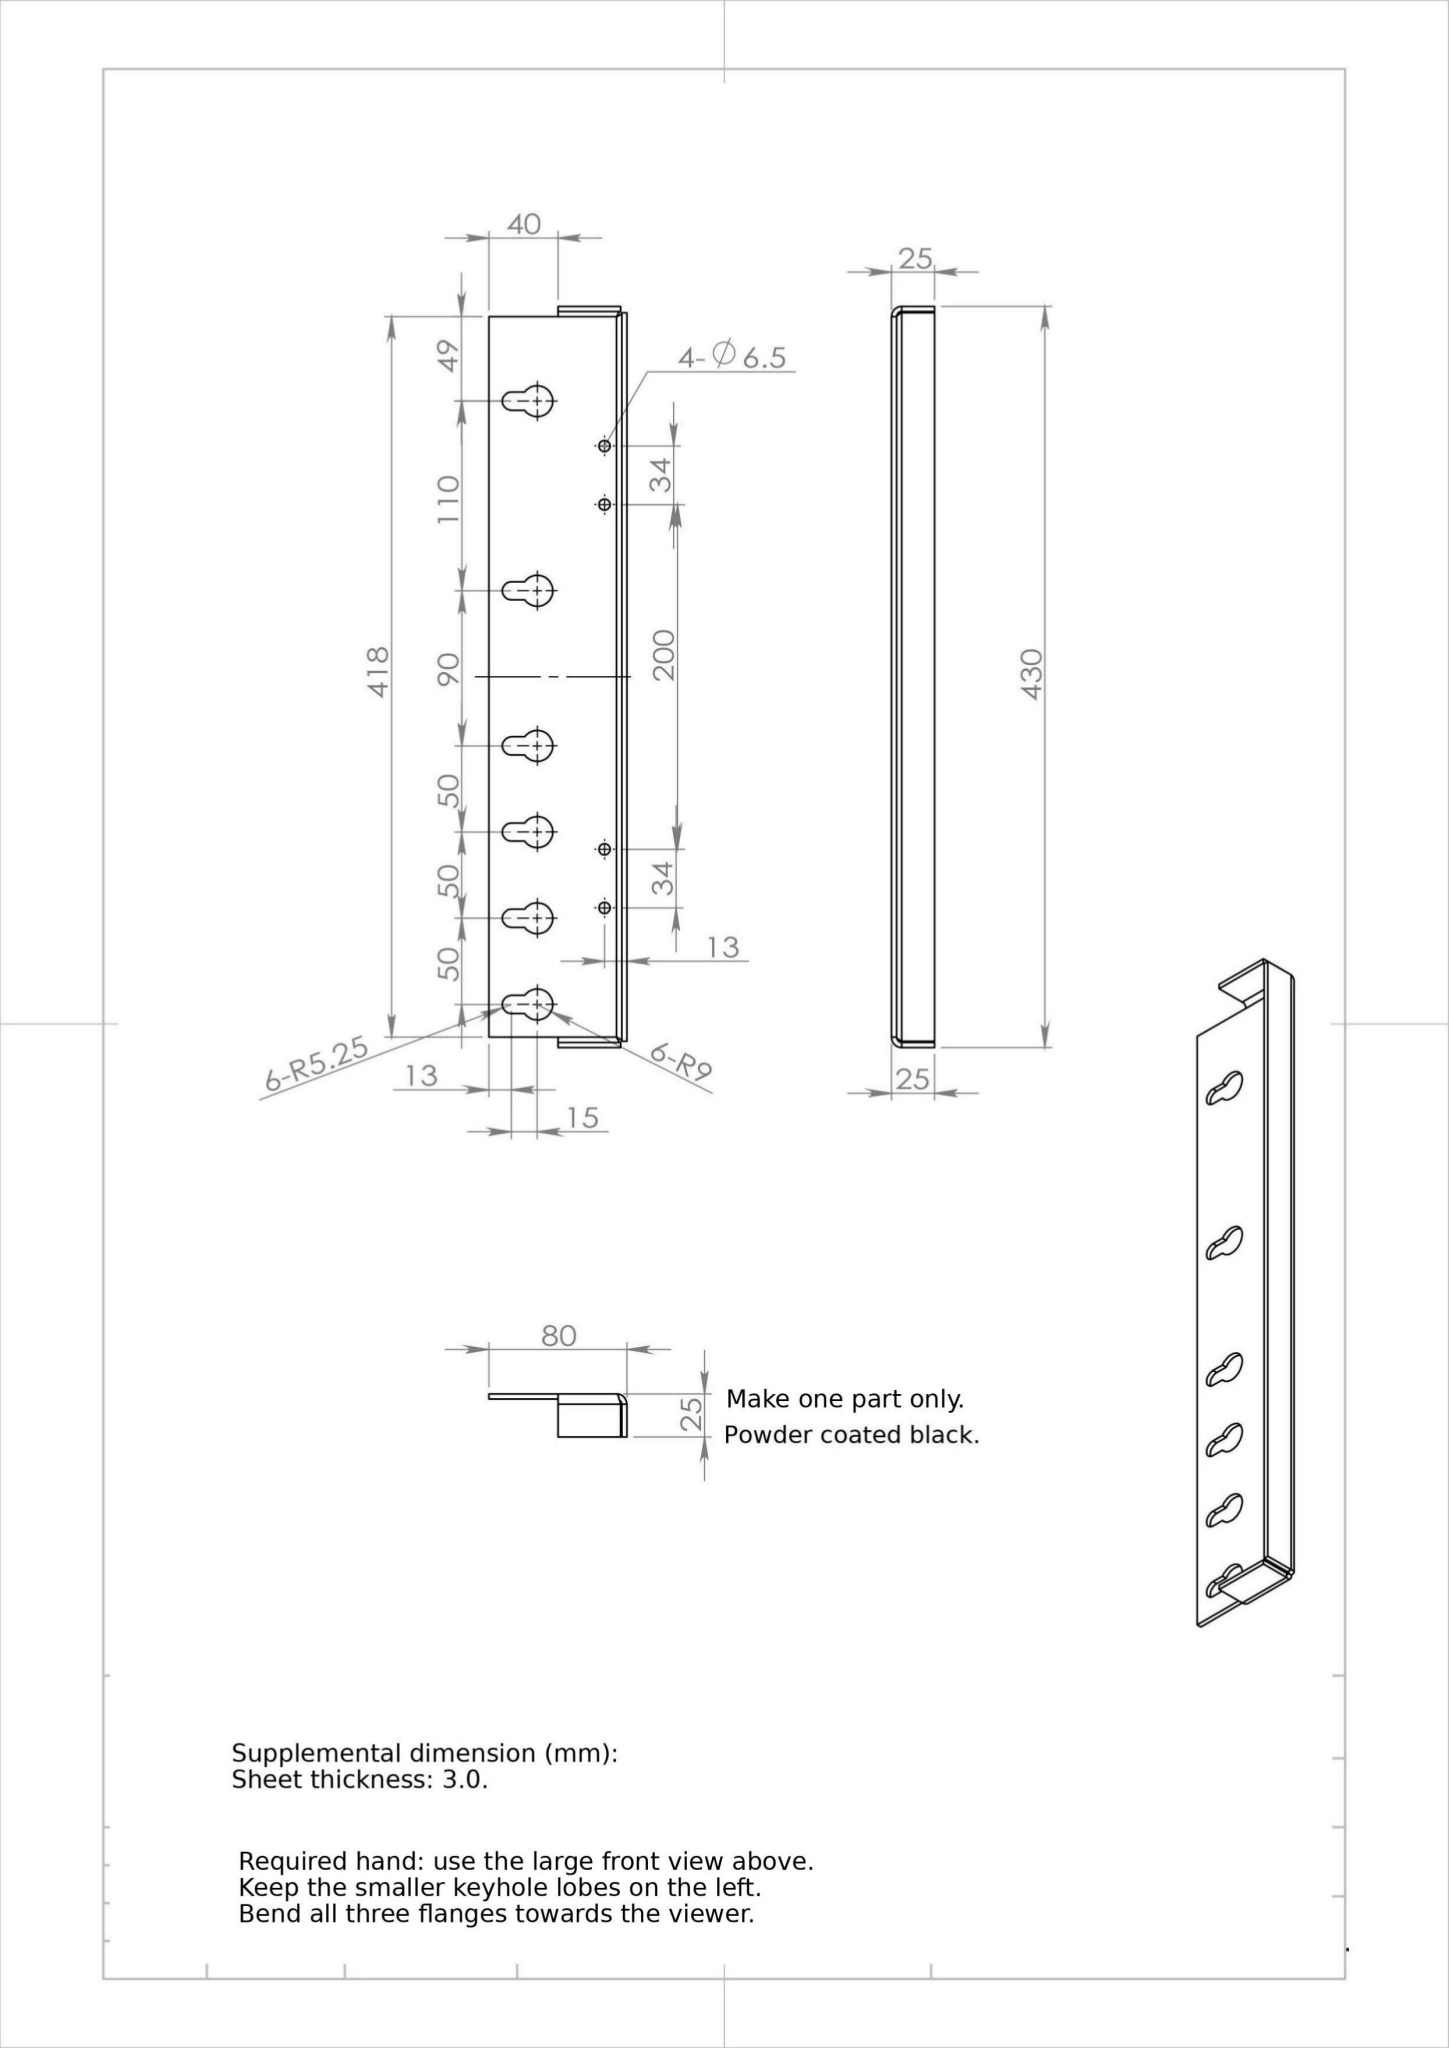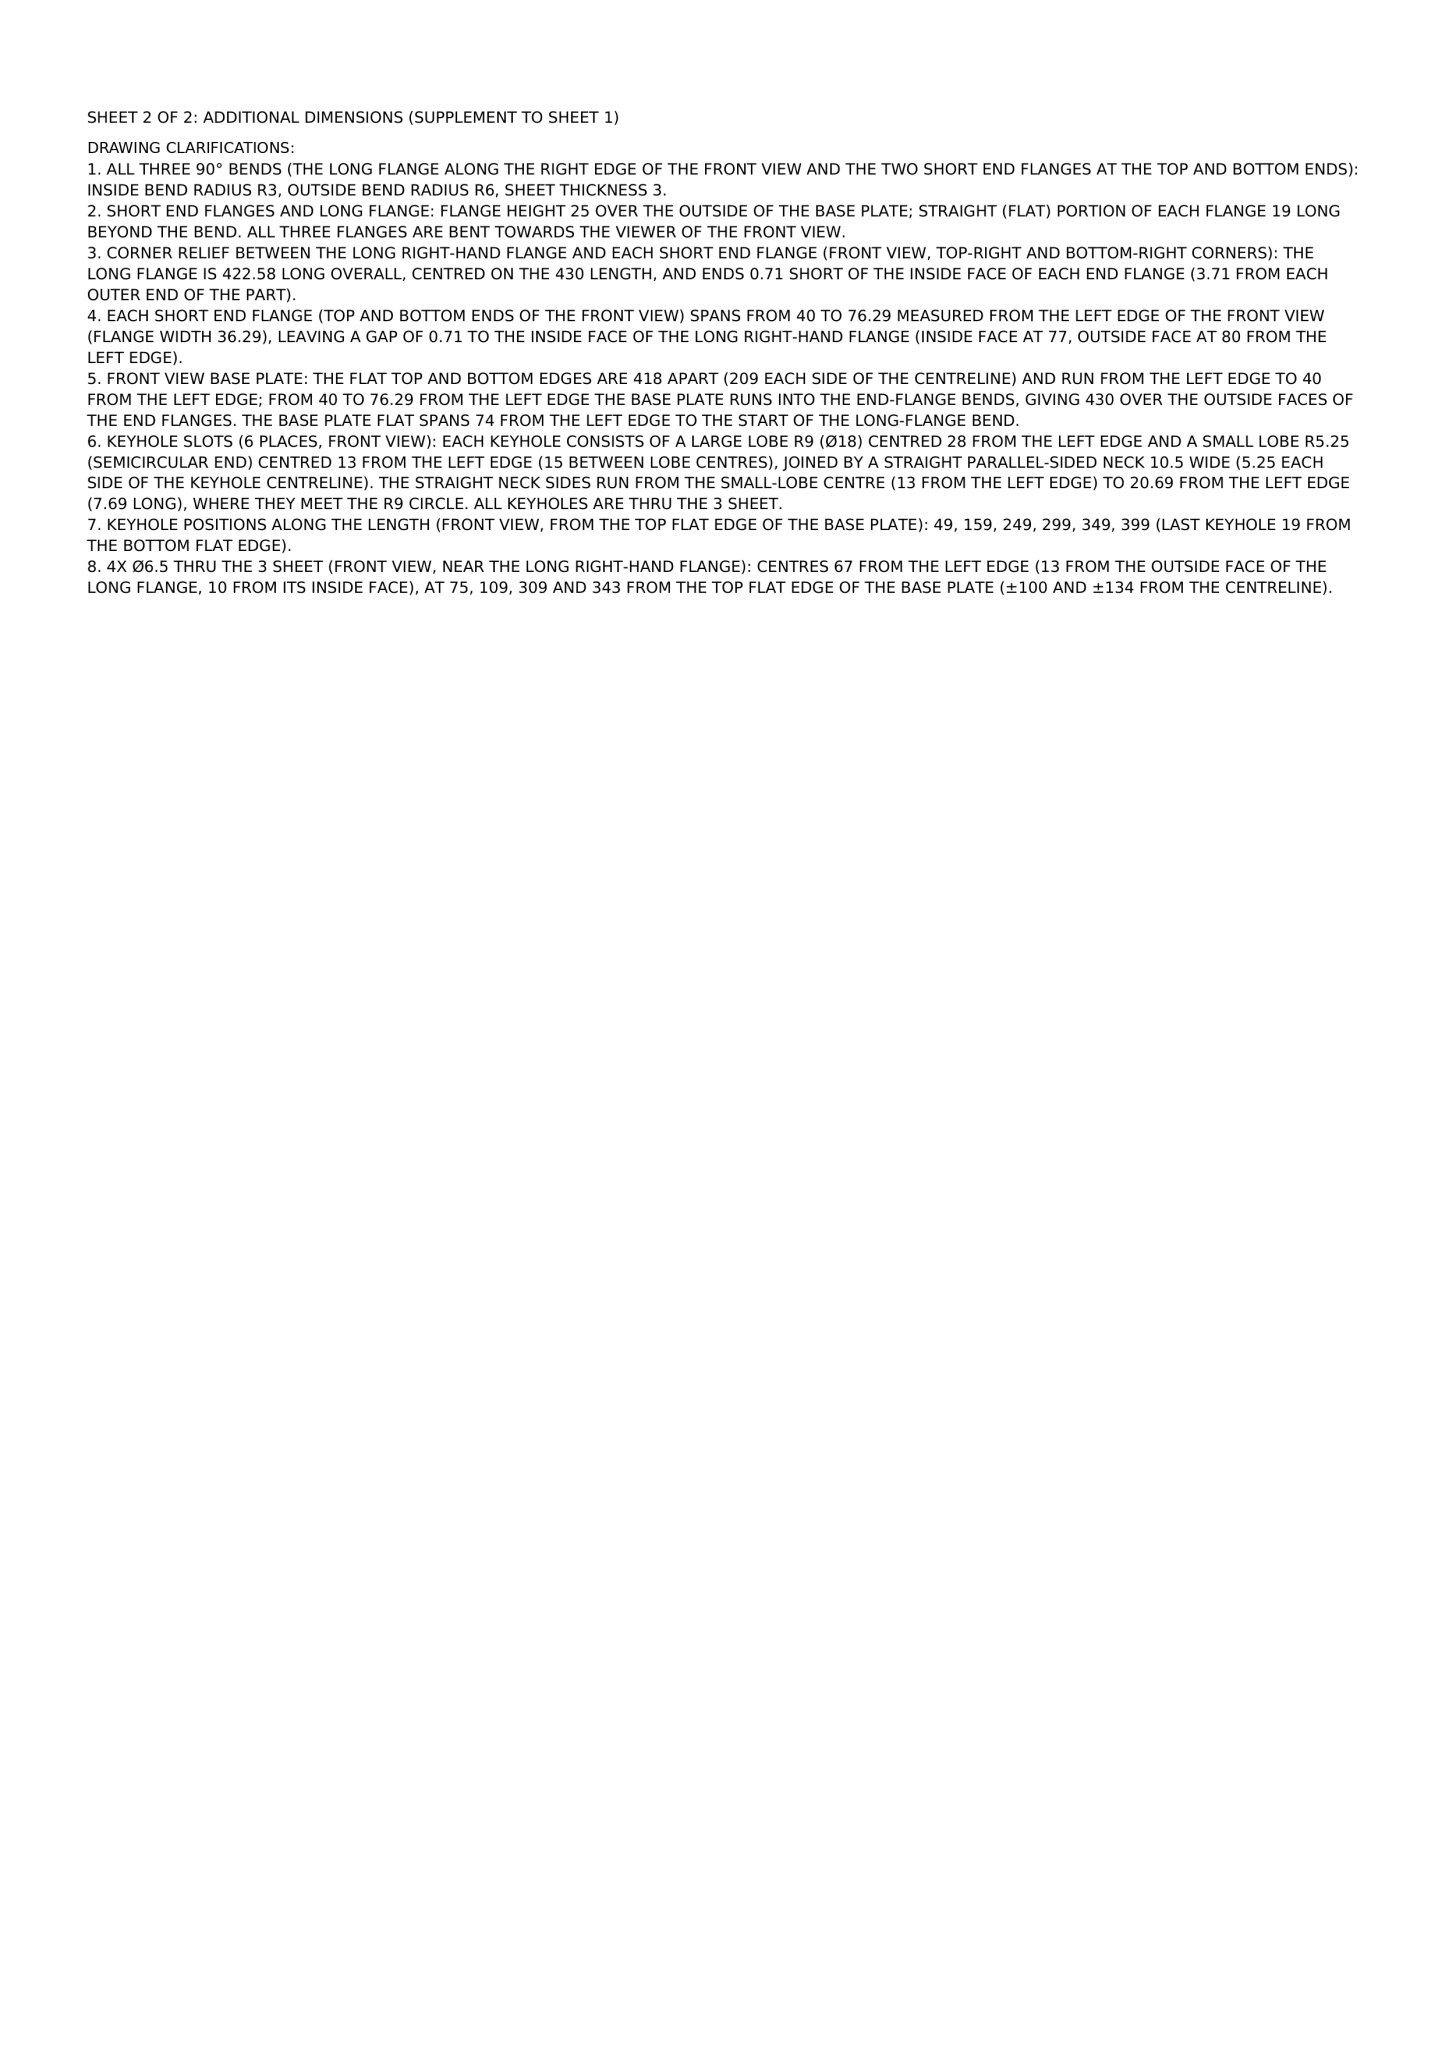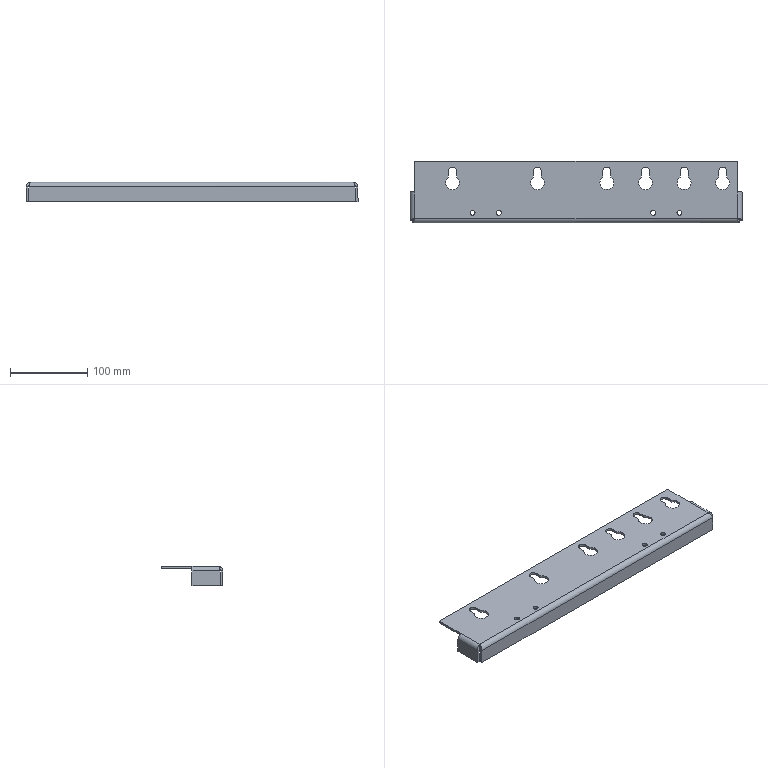Part | NX | mm | 471 | 1 solid | 76 faces | box 430 x 80 x 25 mm | volume 124430 mm3 | cylinder 38 | plane 34 | spline 4 | commonest cylinder face diameters 18 x18 6.5 x8 10.5 x6 12 x3 6 x3